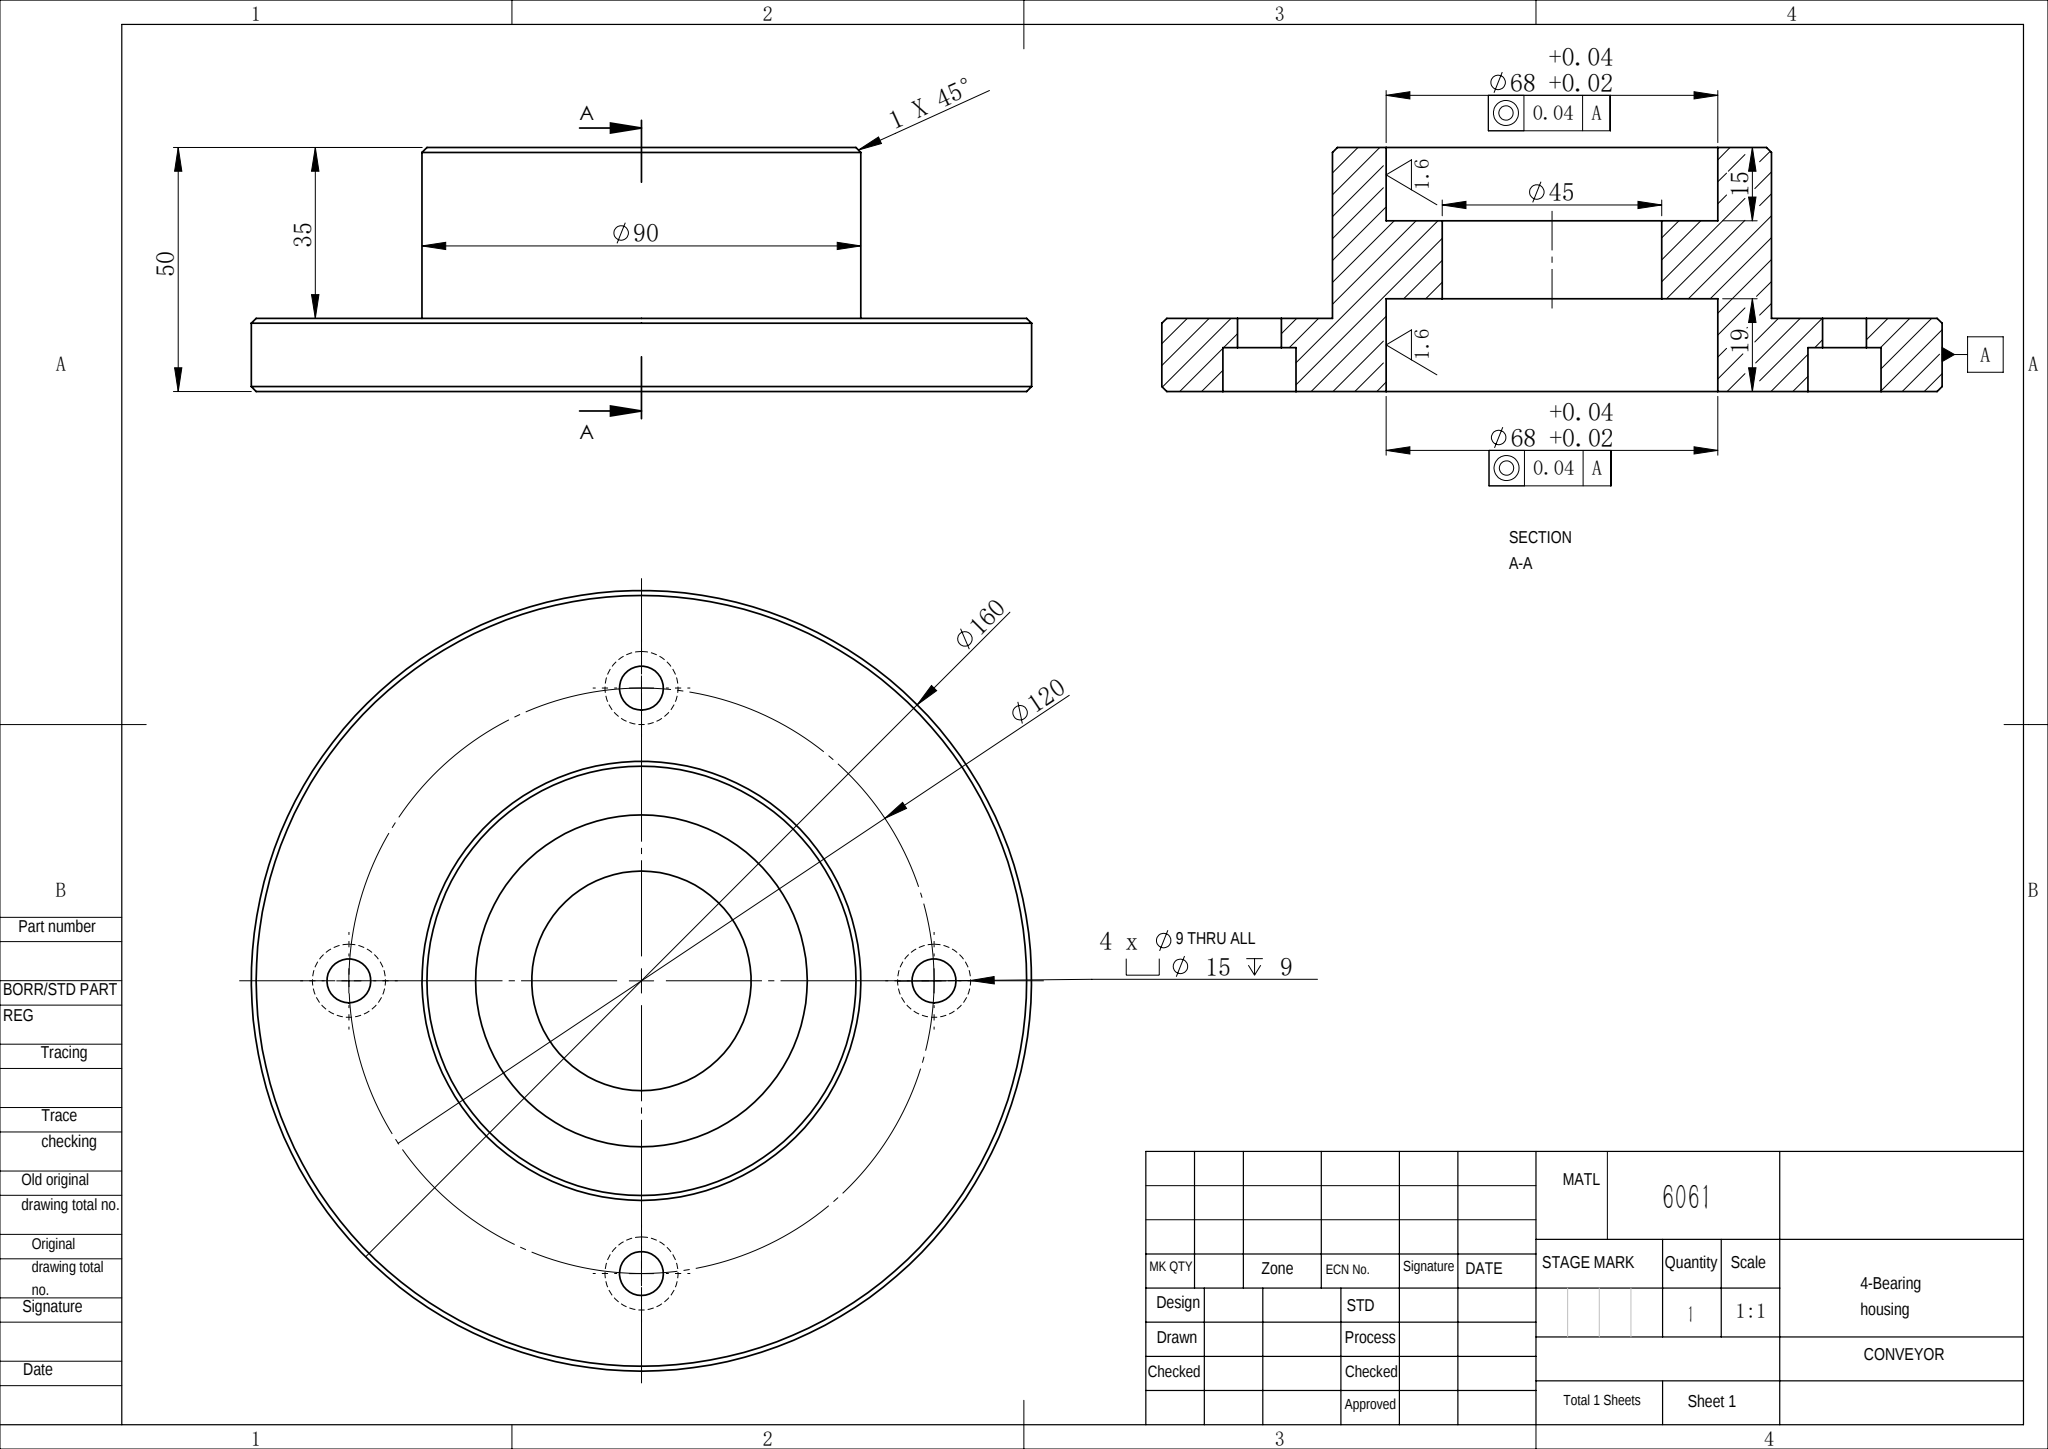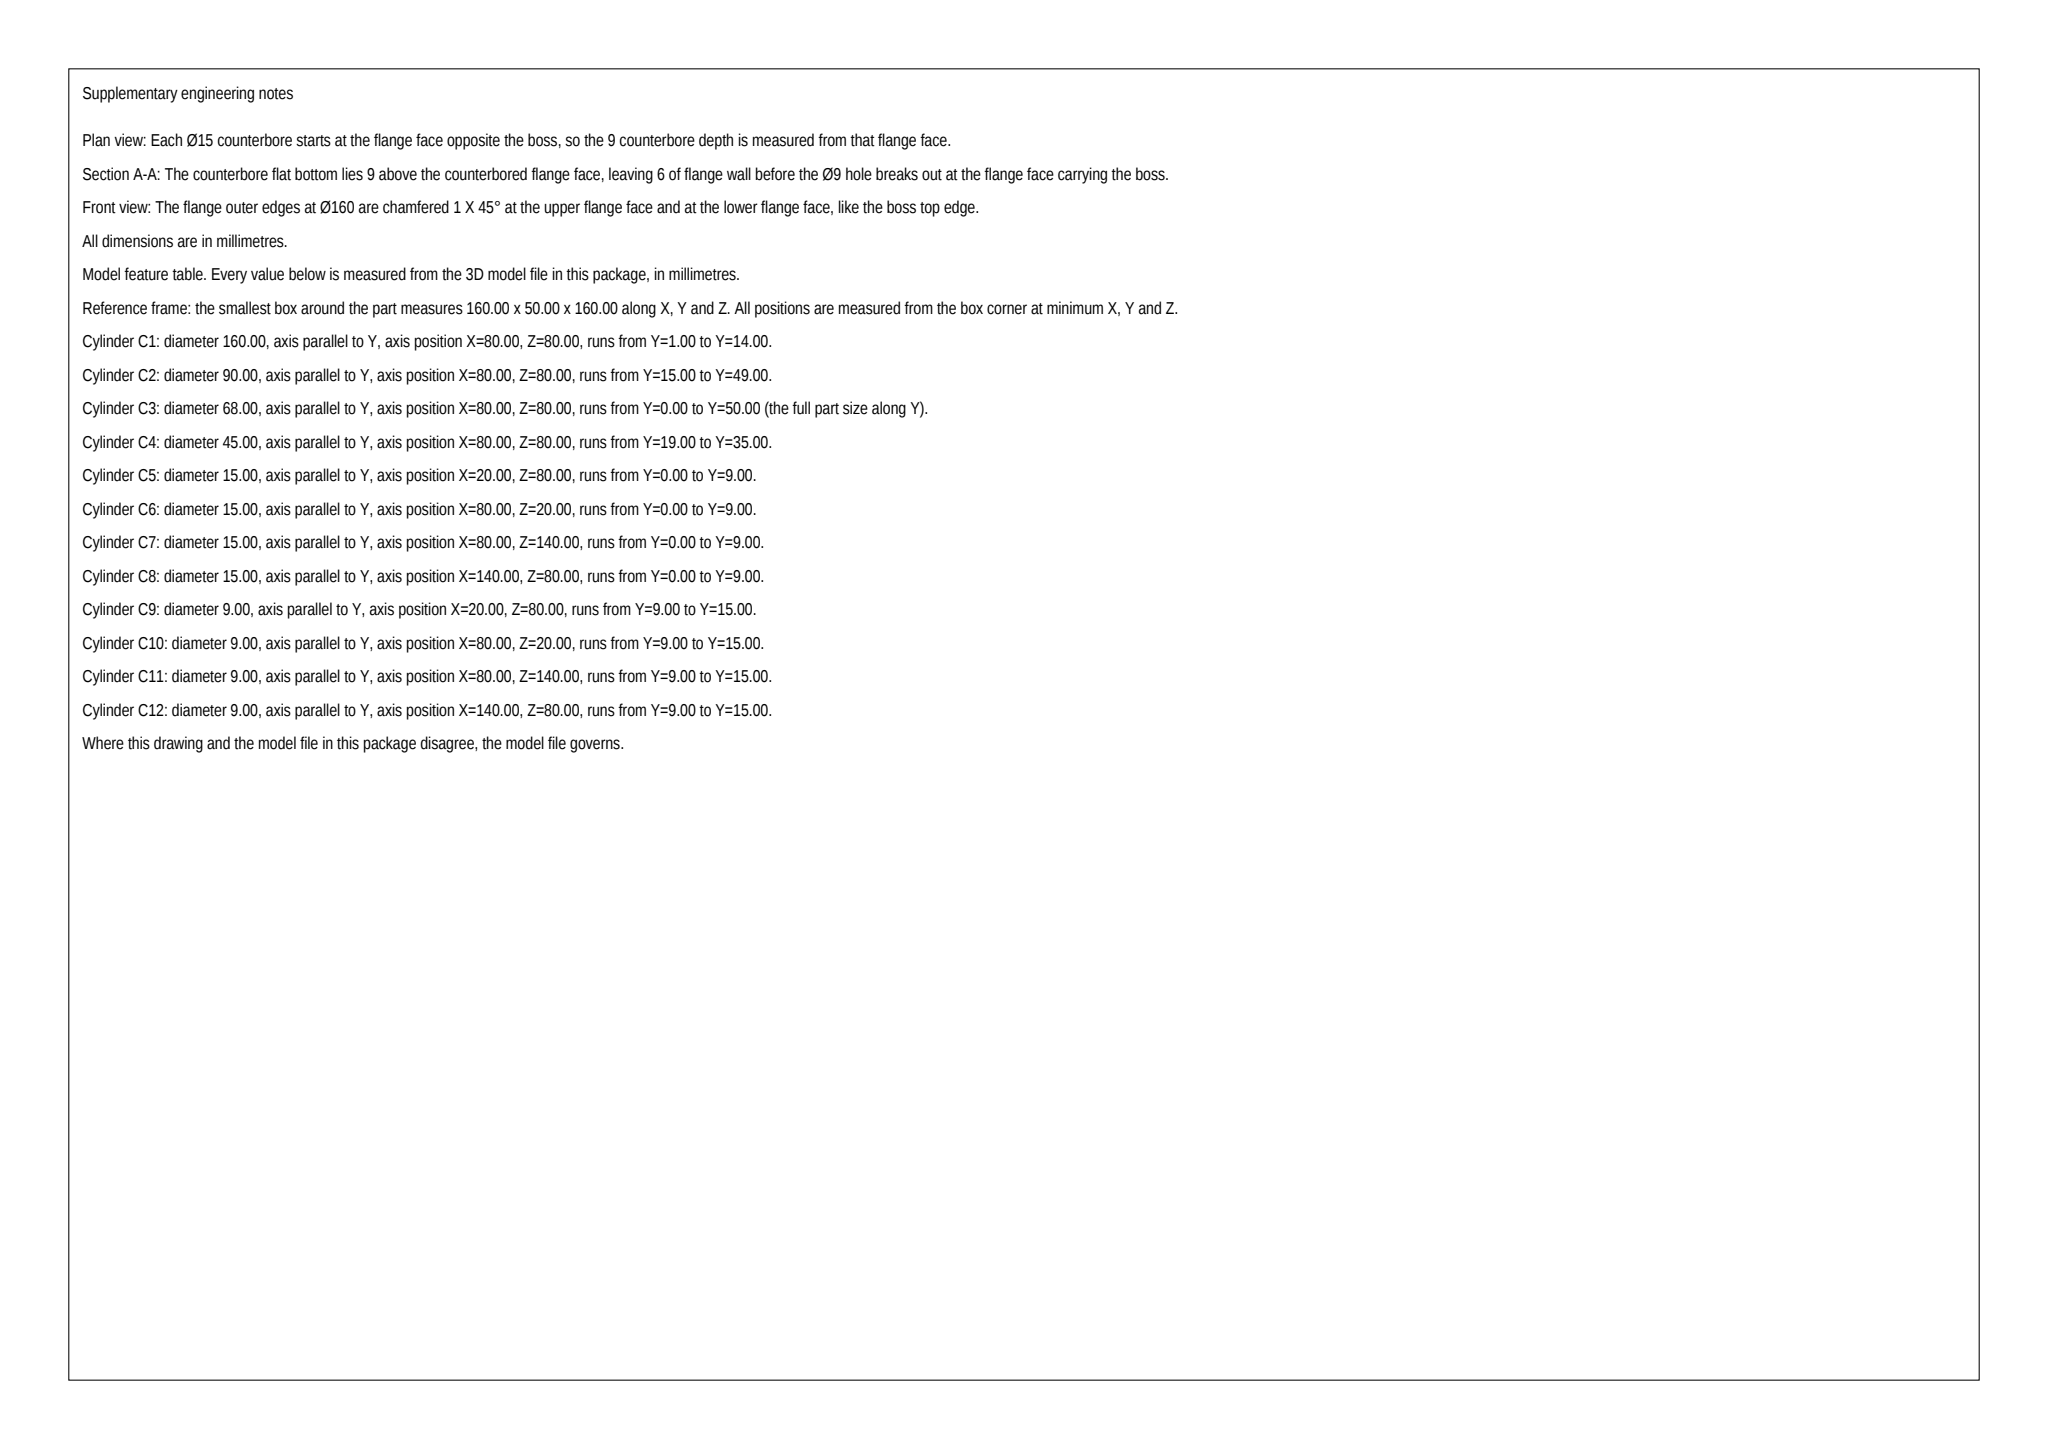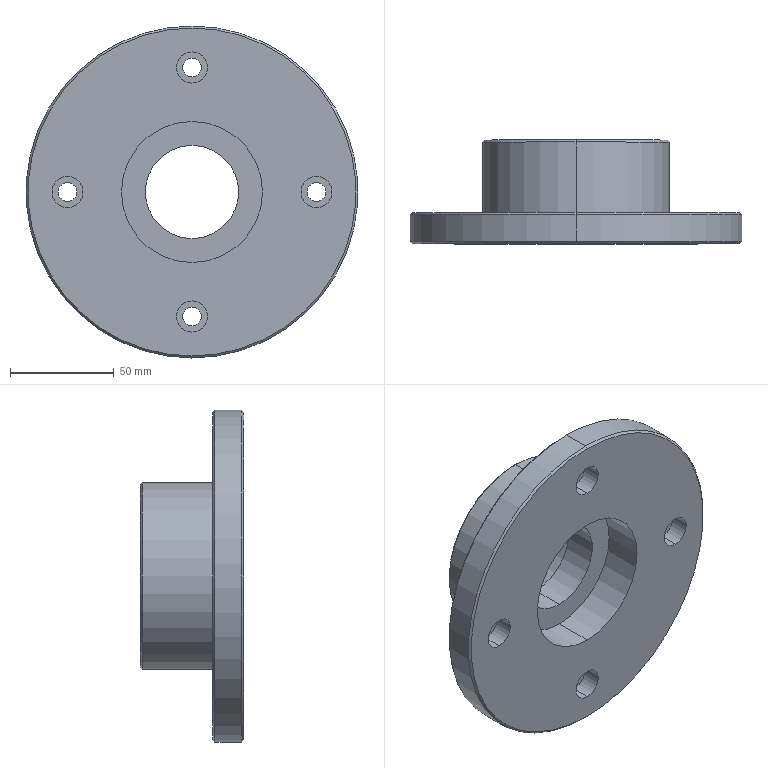Part | SolidWorks | mm | 1 solid | 41 faces | box 160 x 50 x 160 mm | volume 366800 mm3 | cylinder 26 | plane 9 | cone 6 | commonest cylinder face diameters 15 x8 9 x8 68 x4 90 x2 160 x2 45 x2
build123d program:
from build123d import *

# Parameters (mm, degrees)
SKETCH2_R                                         = 34
CUT_EXTRUDE1_DEPTH                                = 15
SKETCH3_R                                         = 22.5
CUT_EXTRUDE2_DEPTH                                = 119.427
CUT_EXTRUDE3_START                                = -19
SKETCH4_R                                         = 34
CUT_EXTRUDE3_DEPTH                                = 19
CHAMFER1_SIZE                                     = 1
HOLE_SIZE_ACCORDING_TO_HEXAGON_SOCKET_D           = 9
HOLE_SIZE_ACCORDING_TO_HEXAGON_SOCKET_CBORE_D     = 15
HOLE_SIZE_ACCORDING_TO_HEXAGON_SOCKET_CBORE_DEPTH = 9


with BuildPart() as part:
    # Sketch1 → Revolve1 (revolve)
    with BuildSketch(Plane.XY, mode=Mode.PRIVATE) as revolve1_sk:
        Polygon((0, 0), (80, 0), (80, 15), (45, 15), (45, 50), (0, 50), align=None)
    revolve(revolve1_sk.sketch.rotate(Axis((0, 0, 0), (0, 1, 0)), 90), axis=Axis((0, 0, 0), (0, 1, 0)))

    # Sketch2 → Cut-Extrude1 (cut)
    with BuildSketch(Plane(origin=(0, 50, 0), x_dir=(1, 0, 0), z_dir=(0, 1, 0))):
        with Locations(Location((0, 0, 0), (0, 0, 270))):
            Circle(SKETCH2_R)
    extrude(amount=-CUT_EXTRUDE1_DEPTH, mode=Mode.SUBTRACT)

    # Sketch3 → Cut-Extrude2 (cut, through all)
    with BuildSketch(Plane(origin=(0, 35, 0), x_dir=(1, 0, 0), z_dir=(0, 1, 0))):
        with Locations(Location((0, 0, 0), (0, 0, 270))):
            Circle(SKETCH3_R)
    extrude(amount=-CUT_EXTRUDE2_DEPTH, mode=Mode.SUBTRACT)

    # Sketch4 → Cut-Extrude3 (cut)
    with BuildSketch(Plane.XZ.offset(CUT_EXTRUDE3_START)):
        with Locations(Location((0, 0, 0), (0, 0, 90))):
            Circle(SKETCH4_R)
    extrude(amount=CUT_EXTRUDE3_DEPTH, mode=Mode.SUBTRACT)

    # Chamfer1
    chamfer1_edges = [part.edges().sort_by_distance(p)[0] for p in [
        (0, 50, 45),
        (0, 15, 80),
        (0, 0, 80),
    ]]
    chamfer(chamfer1_edges, length=CHAMFER1_SIZE)

    # Hole Size _according to_ Hexagon Socket (through all)
    with Locations(Plane(origin=(0, 0, 0), x_dir=(-1, 0, 0), z_dir=(0, -1, 0))):
        with Locations((-60, 0), (60, 0), (0, 60), (0, -60)):
            CounterBoreHole(HOLE_SIZE_ACCORDING_TO_HEXAGON_SOCKET_D / 2, HOLE_SIZE_ACCORDING_TO_HEXAGON_SOCKET_CBORE_D / 2, HOLE_SIZE_ACCORDING_TO_HEXAGON_SOCKET_CBORE_DEPTH)


solid = part.part